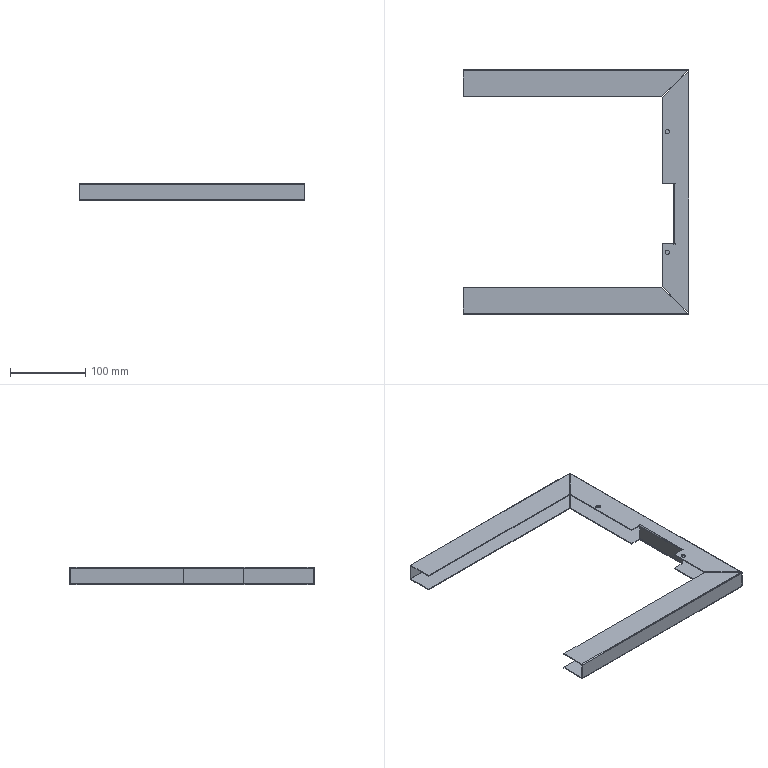Component | SolidWorks | Cover1-8XG1-1 | 1 solid | 98 faces | volume 92917 mm3 | plane 68 | cylinder 22 | spline 8 | commonest cylinder face diameters 0.1 x9 2.5 x9 6 x4